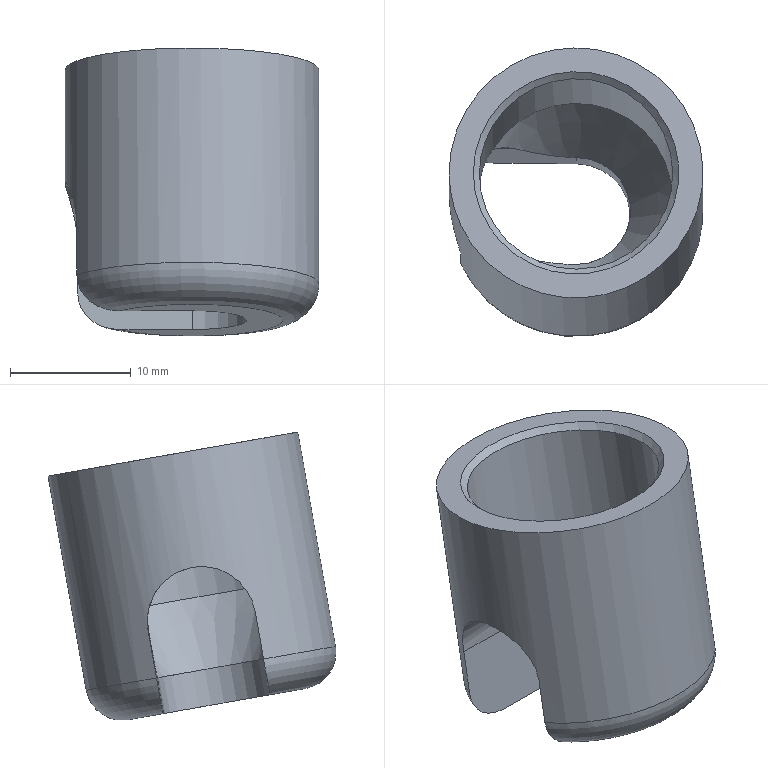Component | NX | BALL_JOINT_OUTER_SLEEVE_2 | 1 solid | 14 faces | volume 3348 mm3 | plane 7 | cylinder 4 | cone 2 | torus 1 | commonest cylinder face diameters 9 x2 21 x1 16 x1